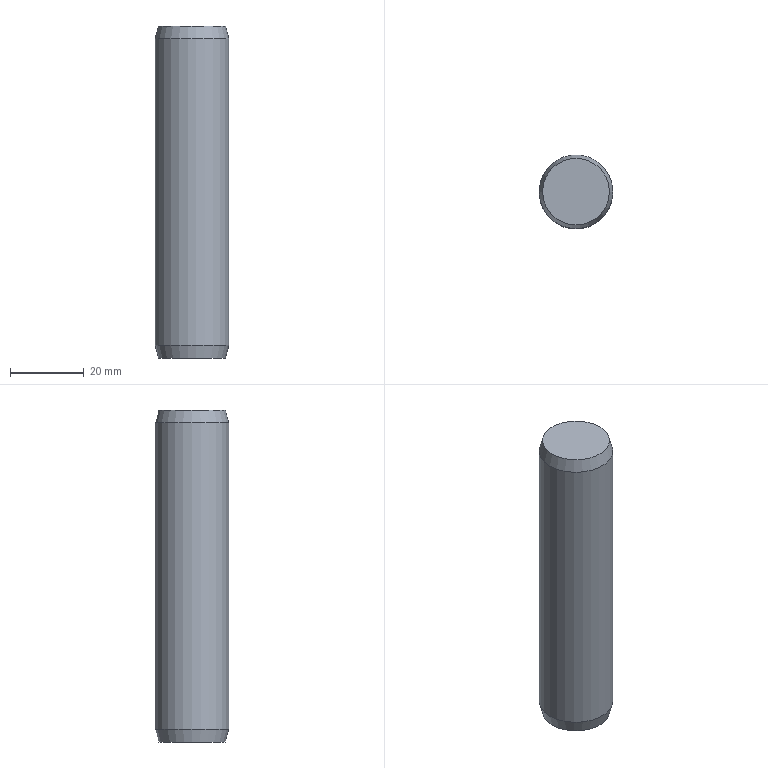Component | NX | GB-T119_1-2000_20X90 | 1 solid | 5 faces | box 20 x 20 x 90 mm | volume 28075 mm3 | plane 2 | cone 2 | cylinder 1 | commonest cylinder face diameters 20 x1
STEP:
#1=CARTESIAN_POINT('',(0.,0.,0.));
#2=DIRECTION('',(0.,0.,1.));
#3=DIRECTION('',(1.,0.,0.));
#4=AXIS2_PLACEMENT_3D('',#1,#2,#3);
#5=CARTESIAN_POINT('',(-129.062,67.5,20.));
#6=VERTEX_POINT('',#5);
#7=CARTESIAN_POINT('',(-120.,67.5,20.));
#8=DIRECTION('',(0.,0.,-1.));
#9=DIRECTION('',(-1.,0.,0.));
#10=AXIS2_PLACEMENT_3D('',#7,#8,#9);
#11=CIRCLE('',#10,9.062);
#12=CARTESIAN_POINT('',(-120.,67.5,20.));
#13=DIRECTION('',(0.,0.,-1.));
#14=DIRECTION('',(-1.,0.,0.));
#15=AXIS2_PLACEMENT_3D('',#12,#13,#14);
#16=PLANE('',#15);
#17=CARTESIAN_POINT('',(0.,0.));
#18=DIRECTION('',(1.,0.));
#19=AXIS2_PLACEMENT_2D('',#17,#18);
#20=CIRCLE('',#19,9.062);
#21=(GEOMETRIC_REPRESENTATION_CONTEXT(2)PARAMETRIC_REPRESENTATION_CONTEXT()REPRESENTATION_CONTEXT('',''));
#22=DEFINITIONAL_REPRESENTATION('',(#20),#21);
#23=PCURVE('',#16,#22);
#24=CARTESIAN_POINT('',(-120.,67.5,20.));
#25=DIRECTION('',(0.,0.,1.));
#26=DIRECTION('',(1.,0.,0.));
#27=AXIS2_PLACEMENT_3D('',#24,#25,#26);
#28=CONICAL_SURFACE('',#27,9.062,0.2618);
#29=CARTESIAN_POINT('',(9.425,-0.));
#30=DIRECTION('',(-1.,0.));
#31=VECTOR('',#30,1.);
#32=LINE('',#29,#31);
#33=(GEOMETRIC_REPRESENTATION_CONTEXT(2)PARAMETRIC_REPRESENTATION_CONTEXT()REPRESENTATION_CONTEXT('',''));
#34=DEFINITIONAL_REPRESENTATION('',(#32),#33);
#35=PCURVE('',#28,#34);
#36=SURFACE_CURVE('',#11,(#23,#35),.PCURVE_S1.);
#37=EDGE_CURVE('',#6,#6,#36,.T.);
#38=ORIENTED_EDGE('',*,*,#37,.T.);
#39=EDGE_LOOP('',(#38));
#40=FACE_BOUND('',#39,.T.);
#41=ADVANCED_FACE('',(#40),#16,.T.);
#42=CARTESIAN_POINT('',(-130.,67.5,23.5));
#43=VERTEX_POINT('',#42);
#44=CARTESIAN_POINT('',(-120.,67.5,23.5));
#45=DIRECTION('',(0.,0.,-1.));
#46=DIRECTION('',(-1.,0.,0.));
#47=AXIS2_PLACEMENT_3D('',#44,#45,#46);
#48=CIRCLE('',#47,10.);
#49=CARTESIAN_POINT('',(9.425,3.5));
#50=DIRECTION('',(-1.,0.));
#51=VECTOR('',#50,1.);
#52=LINE('',#49,#51);
#53=(GEOMETRIC_REPRESENTATION_CONTEXT(2)PARAMETRIC_REPRESENTATION_CONTEXT()REPRESENTATION_CONTEXT('',''));
#54=DEFINITIONAL_REPRESENTATION('',(#52),#53);
#55=PCURVE('',#28,#54);
#56=CARTESIAN_POINT('',(-120.,67.5,110.));
#57=DIRECTION('',(0.,0.,-1.));
#58=DIRECTION('',(-1.,0.,0.));
#59=AXIS2_PLACEMENT_3D('',#56,#57,#58);
#60=CYLINDRICAL_SURFACE('',#59,10.);
#61=CARTESIAN_POINT('',(0.,86.5));
#62=DIRECTION('',(1.,0.));
#63=VECTOR('',#62,1.);
#64=LINE('',#61,#63);
#65=(GEOMETRIC_REPRESENTATION_CONTEXT(2)PARAMETRIC_REPRESENTATION_CONTEXT()REPRESENTATION_CONTEXT('',''));
#66=DEFINITIONAL_REPRESENTATION('',(#64),#65);
#67=PCURVE('',#60,#66);
#68=SURFACE_CURVE('',#48,(#55,#67),.PCURVE_S1.);
#69=EDGE_CURVE('',#43,#43,#68,.T.);
#70=ORIENTED_EDGE('',*,*,#69,.T.);
#71=CARTESIAN_POINT('',(-129.062,67.5,20.));
#72=CARTESIAN_POINT('',(-130.,67.5,23.5));
#73=B_SPLINE_CURVE_WITH_KNOTS('',1,(#71,#72),.UNSPECIFIED.,.F.,.F.,(2,2),(-0.,3.623),.PIECEWISE_BEZIER_KNOTS.);
#74=CARTESIAN_POINT('',(3.142,0.));
#75=DIRECTION('',(0.,1.));
#76=VECTOR('',#75,1.);
#77=LINE('',#74,#76);
#78=(GEOMETRIC_REPRESENTATION_CONTEXT(2)PARAMETRIC_REPRESENTATION_CONTEXT()REPRESENTATION_CONTEXT('',''));
#79=DEFINITIONAL_REPRESENTATION('',(#77),#78);
#80=PCURVE('',#28,#79);
#81=CARTESIAN_POINT('',(9.425,0.));
#82=DIRECTION('',(0.,1.));
#83=VECTOR('',#82,1.);
#84=LINE('',#81,#83);
#85=(GEOMETRIC_REPRESENTATION_CONTEXT(2)PARAMETRIC_REPRESENTATION_CONTEXT()REPRESENTATION_CONTEXT('',''));
#86=DEFINITIONAL_REPRESENTATION('',(#84),#85);
#87=PCURVE('',#28,#86);
#88=SEAM_CURVE('',#73,(#80,#87),.PCURVE_S1.);
#89=EDGE_CURVE('',#6,#43,#88,.T.);
#90=ORIENTED_EDGE('',*,*,#89,.F.);
#91=ORIENTED_EDGE('',*,*,#37,.F.);
#92=ORIENTED_EDGE('',*,*,#89,.T.);
#93=EDGE_LOOP('',(#70,#90,#91,#92));
#94=FACE_BOUND('',#93,.T.);
#95=ADVANCED_FACE('',(#94),#28,.T.);
#96=CARTESIAN_POINT('',(-130.,67.5,106.5));
#97=VERTEX_POINT('',#96);
#98=CARTESIAN_POINT('',(-120.,67.5,106.5));
#99=DIRECTION('',(0.,0.,-1.));
#100=DIRECTION('',(-1.,0.,0.));
#101=AXIS2_PLACEMENT_3D('',#98,#99,#100);
#102=CIRCLE('',#101,10.);
#103=CARTESIAN_POINT('',(0.,3.5));
#104=DIRECTION('',(1.,0.));
#105=VECTOR('',#104,1.);
#106=LINE('',#103,#105);
#107=(GEOMETRIC_REPRESENTATION_CONTEXT(2)PARAMETRIC_REPRESENTATION_CONTEXT()REPRESENTATION_CONTEXT('',''));
#108=DEFINITIONAL_REPRESENTATION('',(#106),#107);
#109=PCURVE('',#60,#108);
#110=CARTESIAN_POINT('',(-120.,67.5,106.5));
#111=DIRECTION('',(0.,0.,-1.));
#112=DIRECTION('',(-1.,0.,0.));
#113=AXIS2_PLACEMENT_3D('',#110,#111,#112);
#114=CONICAL_SURFACE('',#113,10.,0.2618);
#115=CARTESIAN_POINT('',(0.,0.));
#116=DIRECTION('',(1.,0.));
#117=VECTOR('',#116,1.);
#118=LINE('',#115,#117);
#119=(GEOMETRIC_REPRESENTATION_CONTEXT(2)PARAMETRIC_REPRESENTATION_CONTEXT()REPRESENTATION_CONTEXT('',''));
#120=DEFINITIONAL_REPRESENTATION('',(#118),#119);
#121=PCURVE('',#114,#120);
#122=SURFACE_CURVE('',#102,(#109,#121),.PCURVE_S1.);
#123=EDGE_CURVE('',#97,#97,#122,.T.);
#124=ORIENTED_EDGE('',*,*,#123,.T.);
#125=CARTESIAN_POINT('',(-130.,67.5,106.5));
#126=CARTESIAN_POINT('',(-130.,67.5,23.5));
#127=B_SPLINE_CURVE_WITH_KNOTS('',1,(#125,#126),.UNSPECIFIED.,.F.,.F.,(2,2),(3.5,86.5),.PIECEWISE_BEZIER_KNOTS.);
#128=CARTESIAN_POINT('',(6.283,0.));
#129=DIRECTION('',(0.,1.));
#130=VECTOR('',#129,1.);
#131=LINE('',#128,#130);
#132=(GEOMETRIC_REPRESENTATION_CONTEXT(2)PARAMETRIC_REPRESENTATION_CONTEXT()REPRESENTATION_CONTEXT('',''));
#133=DEFINITIONAL_REPRESENTATION('',(#131),#132);
#134=PCURVE('',#60,#133);
#135=CARTESIAN_POINT('',(0.,0.));
#136=DIRECTION('',(0.,1.));
#137=VECTOR('',#136,1.);
#138=LINE('',#135,#137);
#139=(GEOMETRIC_REPRESENTATION_CONTEXT(2)PARAMETRIC_REPRESENTATION_CONTEXT()REPRESENTATION_CONTEXT('',''));
#140=DEFINITIONAL_REPRESENTATION('',(#138),#139);
#141=PCURVE('',#60,#140);
#142=SEAM_CURVE('',#127,(#134,#141),.PCURVE_S1.);
#143=EDGE_CURVE('',#97,#43,#142,.T.);
#144=ORIENTED_EDGE('',*,*,#143,.T.);
#145=ORIENTED_EDGE('',*,*,#69,.F.);
#146=ORIENTED_EDGE('',*,*,#143,.F.);
#147=EDGE_LOOP('',(#124,#144,#145,#146));
#148=FACE_BOUND('',#147,.T.);
#149=ADVANCED_FACE('',(#148),#60,.T.);
#150=CARTESIAN_POINT('',(-129.062,67.5,110.));
#151=VERTEX_POINT('',#150);
#152=CARTESIAN_POINT('',(-120.,67.5,110.));
#153=DIRECTION('',(0.,0.,-1.));
#154=DIRECTION('',(-1.,0.,0.));
#155=AXIS2_PLACEMENT_3D('',#152,#153,#154);
#156=CIRCLE('',#155,9.062);
#157=CARTESIAN_POINT('',(0.,-3.5));
#158=DIRECTION('',(1.,0.));
#159=VECTOR('',#158,1.);
#160=LINE('',#157,#159);
#161=(GEOMETRIC_REPRESENTATION_CONTEXT(2)PARAMETRIC_REPRESENTATION_CONTEXT()REPRESENTATION_CONTEXT('',''));
#162=DEFINITIONAL_REPRESENTATION('',(#160),#161);
#163=PCURVE('',#114,#162);
#164=CARTESIAN_POINT('',(-110.938,67.5,110.));
#165=DIRECTION('',(0.,0.,1.));
#166=DIRECTION('',(1.,0.,0.));
#167=AXIS2_PLACEMENT_3D('',#164,#165,#166);
#168=PLANE('',#167);
#169=CARTESIAN_POINT('',(-18.124,0.));
#170=CARTESIAN_POINT('',(-18.124,15.696));
#171=CARTESIAN_POINT('',(-4.531,7.848));
#172=CARTESIAN_POINT('',(9.062,0.));
#173=CARTESIAN_POINT('',(-4.531,-7.848));
#174=CARTESIAN_POINT('',(-18.124,-15.696));
#175=CARTESIAN_POINT('',(-18.124,0.));
#176=(BOUNDED_CURVE()B_SPLINE_CURVE(2,(#169,#170,#171,#172,#173,#174,#175),.UNSPECIFIED.,.T.,.F.)B_SPLINE_CURVE_WITH_KNOTS((1,2,2,2,2,1),(-2.094,0.,2.094,4.189,6.283,8.378),.UNSPECIFIED.)CURVE()GEOMETRIC_REPRESENTATION_ITEM()RATIONAL_B_SPLINE_CURVE((1.,0.5,1.,0.5,1.,0.5,1.))REPRESENTATION_ITEM(''));
#177=(GEOMETRIC_REPRESENTATION_CONTEXT(2)PARAMETRIC_REPRESENTATION_CONTEXT()REPRESENTATION_CONTEXT('',''));
#178=DEFINITIONAL_REPRESENTATION('',(#176),#177);
#179=PCURVE('',#168,#178);
#180=SURFACE_CURVE('',#156,(#163,#179),.PCURVE_S1.);
#181=EDGE_CURVE('',#151,#151,#180,.T.);
#182=ORIENTED_EDGE('',*,*,#181,.T.);
#183=CARTESIAN_POINT('',(-129.062,67.5,110.));
#184=CARTESIAN_POINT('',(-130.,67.5,106.5));
#185=B_SPLINE_CURVE_WITH_KNOTS('',1,(#183,#184),.UNSPECIFIED.,.F.,.F.,(2,2),(-3.623,0.),.PIECEWISE_BEZIER_KNOTS.);
#186=CARTESIAN_POINT('',(6.283,0.));
#187=DIRECTION('',(0.,1.));
#188=VECTOR('',#187,1.);
#189=LINE('',#186,#188);
#190=(GEOMETRIC_REPRESENTATION_CONTEXT(2)PARAMETRIC_REPRESENTATION_CONTEXT()REPRESENTATION_CONTEXT('',''));
#191=DEFINITIONAL_REPRESENTATION('',(#189),#190);
#192=PCURVE('',#114,#191);
#193=CARTESIAN_POINT('',(0.,0.));
#194=DIRECTION('',(0.,1.));
#195=VECTOR('',#194,1.);
#196=LINE('',#193,#195);
#197=(GEOMETRIC_REPRESENTATION_CONTEXT(2)PARAMETRIC_REPRESENTATION_CONTEXT()REPRESENTATION_CONTEXT('',''));
#198=DEFINITIONAL_REPRESENTATION('',(#196),#197);
#199=PCURVE('',#114,#198);
#200=SEAM_CURVE('',#185,(#192,#199),.PCURVE_S1.);
#201=EDGE_CURVE('',#151,#97,#200,.T.);
#202=ORIENTED_EDGE('',*,*,#201,.T.);
#203=ORIENTED_EDGE('',*,*,#123,.F.);
#204=ORIENTED_EDGE('',*,*,#201,.F.);
#205=EDGE_LOOP('',(#182,#202,#203,#204));
#206=FACE_BOUND('',#205,.T.);
#207=ADVANCED_FACE('',(#206),#114,.T.);
#208=ORIENTED_EDGE('',*,*,#181,.F.);
#209=EDGE_LOOP('',(#208));
#210=FACE_BOUND('',#209,.T.);
#211=ADVANCED_FACE('',(#210),#168,.T.);
#212=CLOSED_SHELL('',(#41,#95,#149,#207,#211));
#213=MANIFOLD_SOLID_BREP('',#212);
#214=(LENGTH_UNIT()NAMED_UNIT(*)SI_UNIT(.MILLI.,.METRE.));
#215=UNCERTAINTY_MEASURE_WITH_UNIT(LENGTH_MEASURE(0.00001),#214,'','');
#216=(NAMED_UNIT(*)PLANE_ANGLE_UNIT()SI_UNIT($,.RADIAN.));
#217=(NAMED_UNIT(*)SI_UNIT($,.STERADIAN.)SOLID_ANGLE_UNIT());
#218=(GEOMETRIC_REPRESENTATION_CONTEXT(3)GLOBAL_UNCERTAINTY_ASSIGNED_CONTEXT((#215))GLOBAL_UNIT_ASSIGNED_CONTEXT((#214,#216,#217))REPRESENTATION_CONTEXT('',''));
#219=ADVANCED_BREP_SHAPE_REPRESENTATION('',(#4,#213),#218);